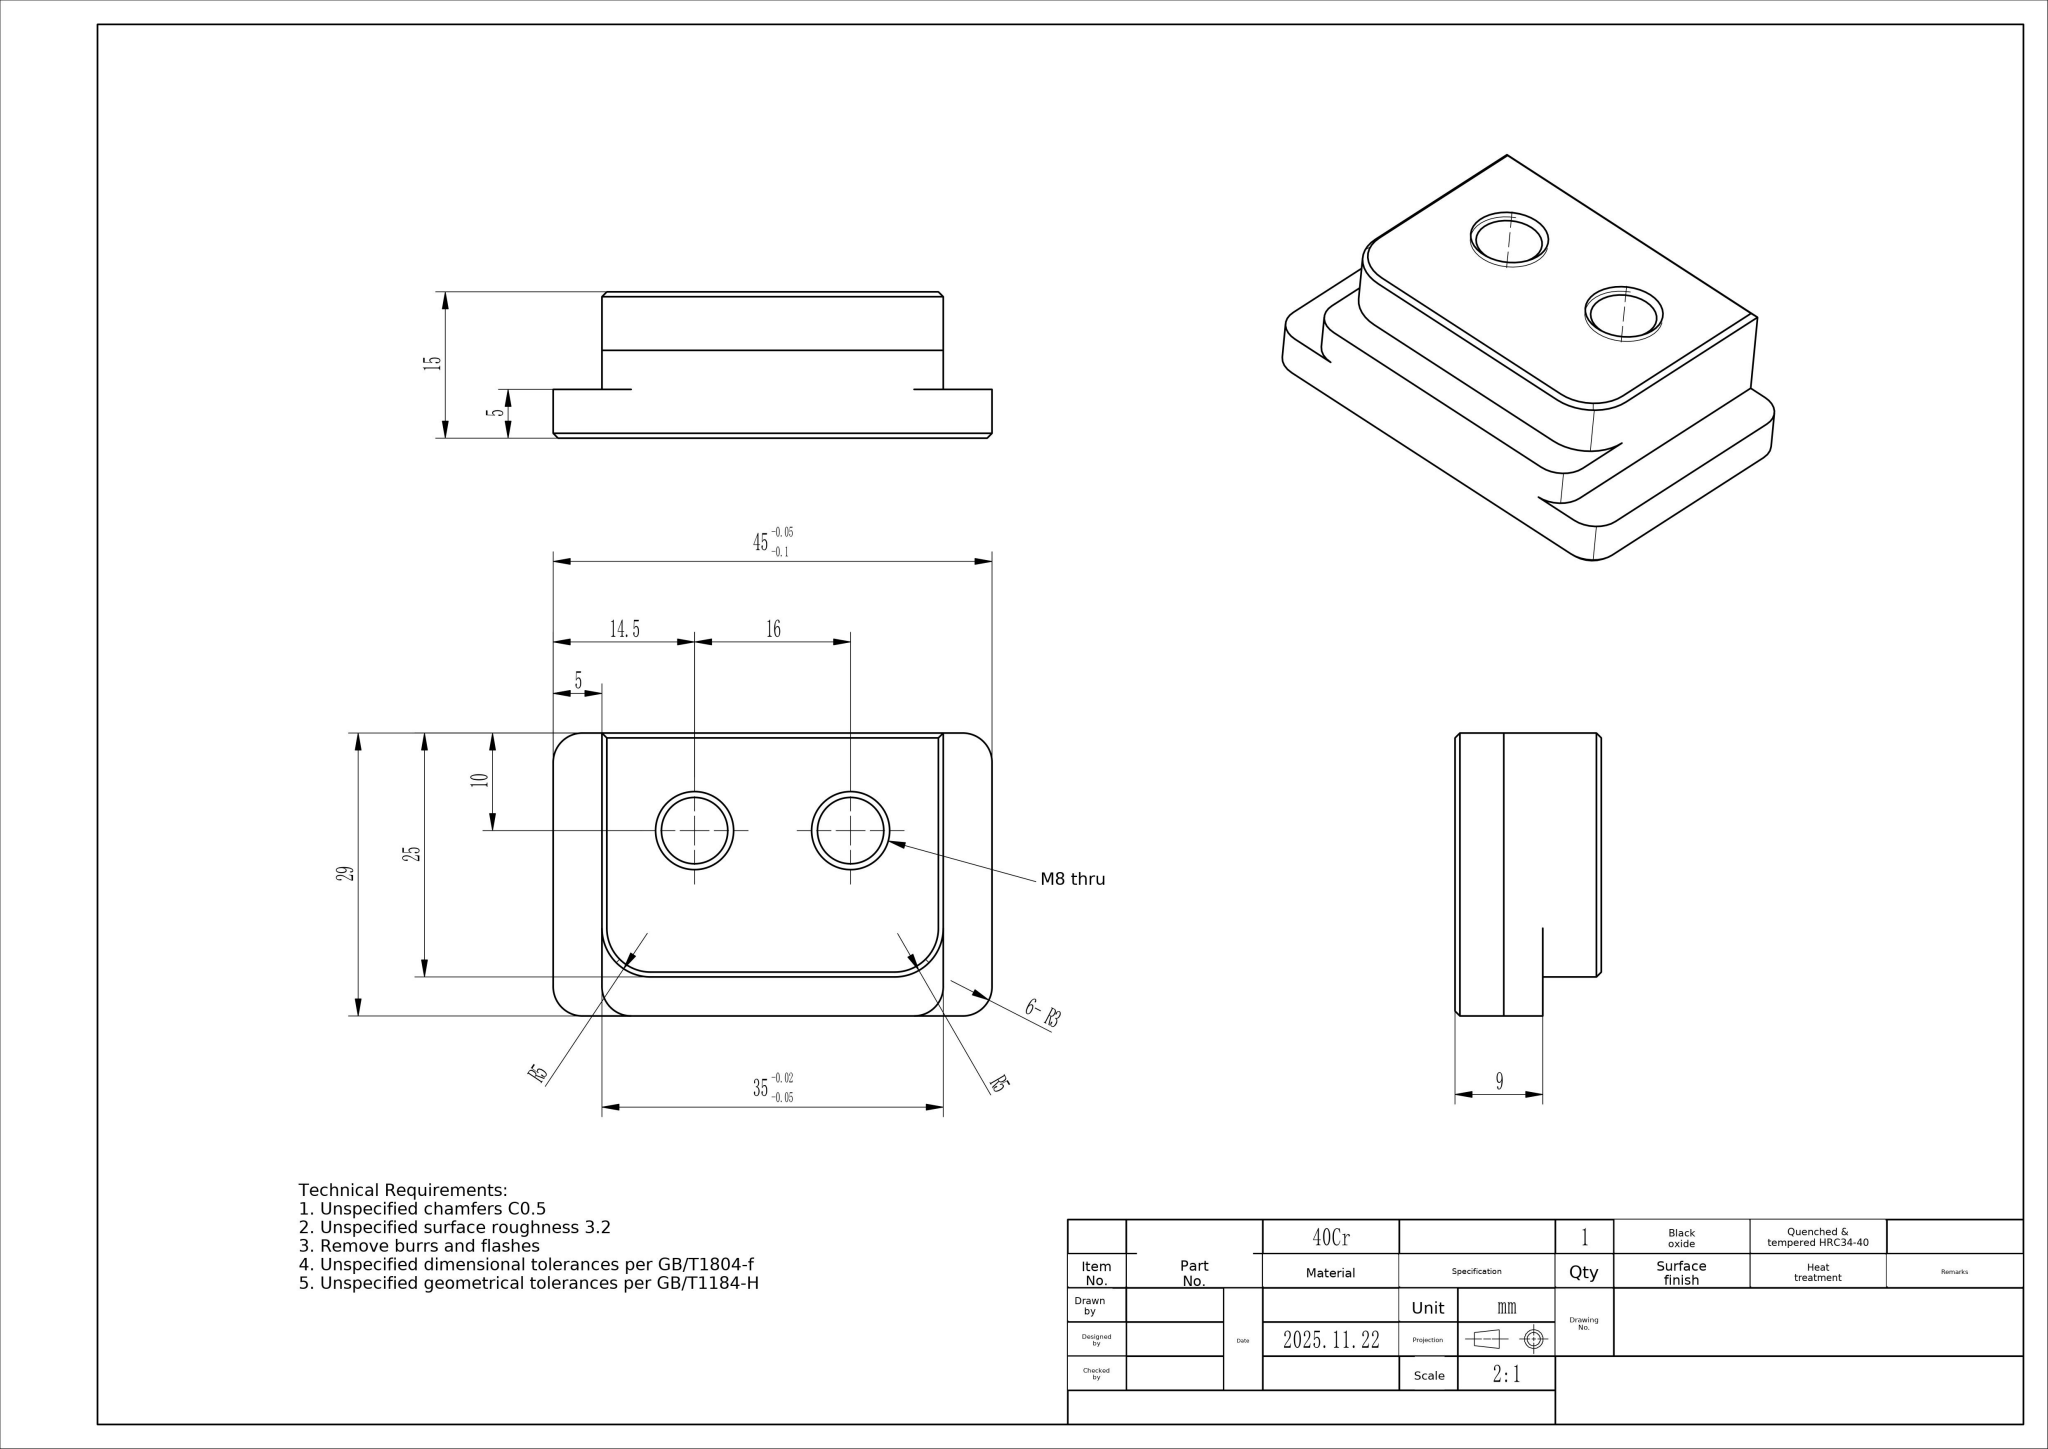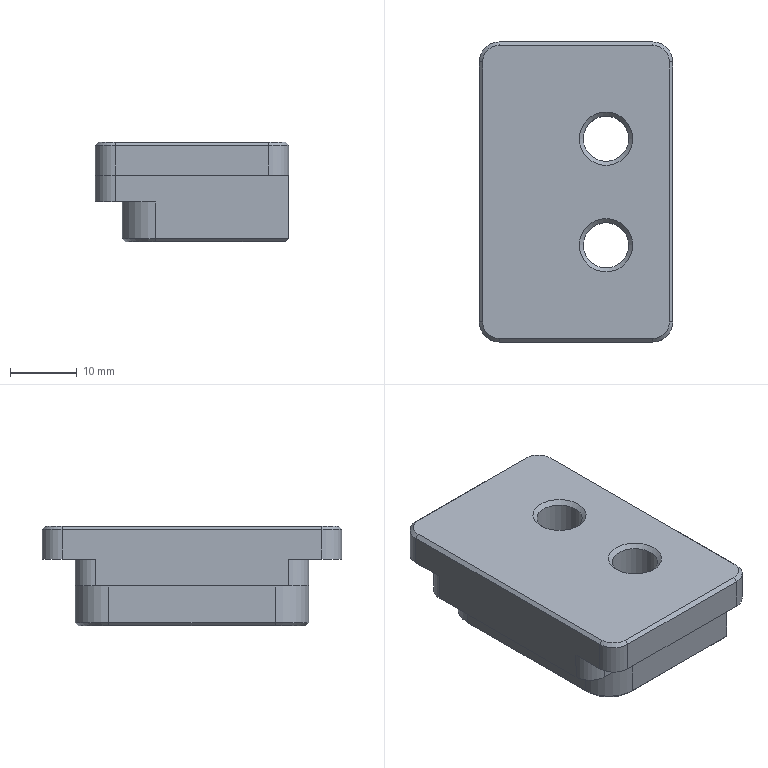Part | NX | mm | 1 solid | 40 faces | box 29 x 45 x 15 mm | volume 14579 mm3 | plane 20 | cylinder 10 | cone 10 | commonest cylinder face diameters 6 x6 6.8 x2 10 x2